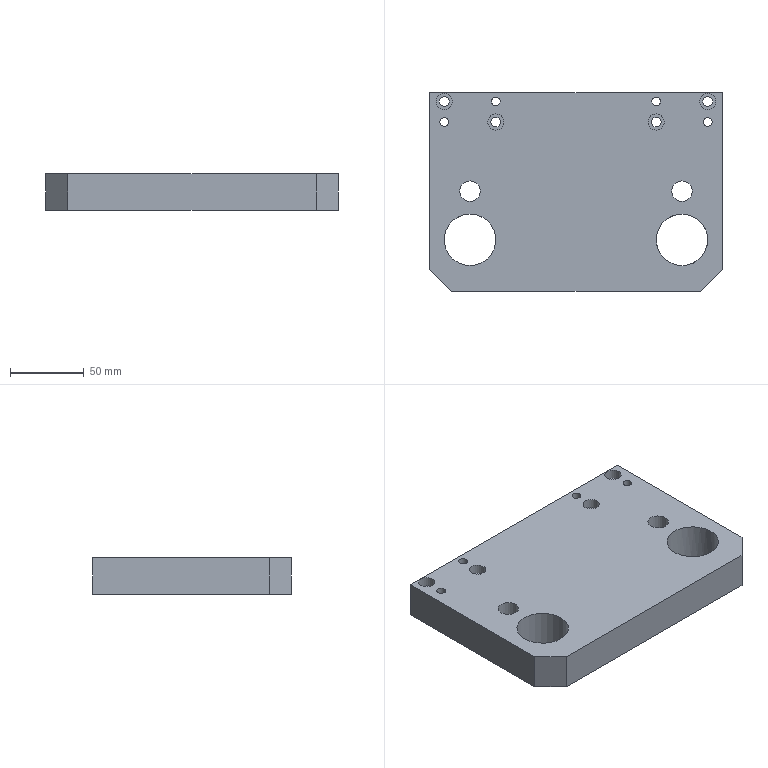Component | NX | DRILL_TEMPLATE | 1 solid | 28 faces | volume 602294 mm3 | cylinder 16 | plane 12 | commonest cylinder face diameters 6 x4 6.6 x4 11 x4 35 x2 14 x2